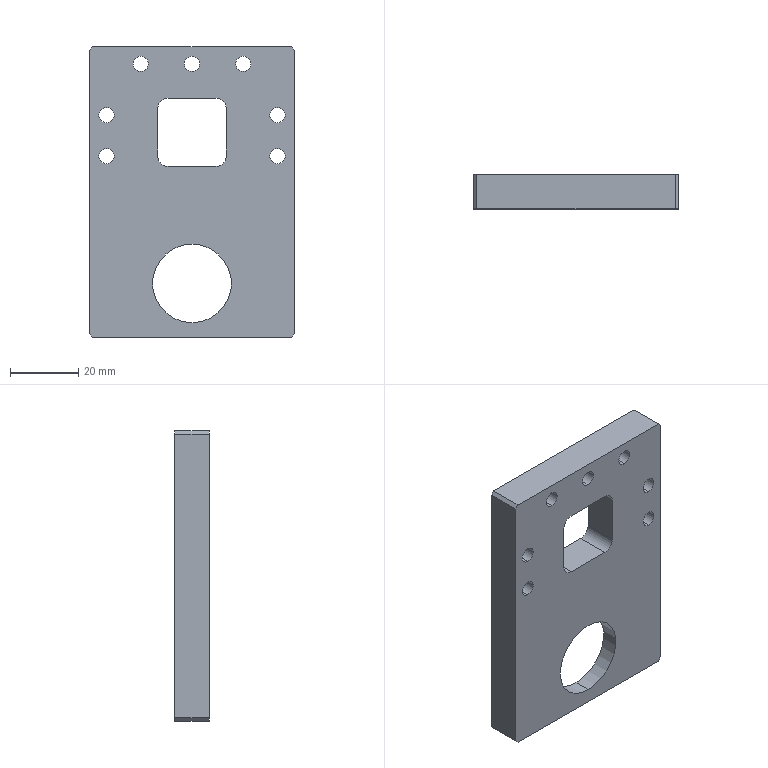Component | SolidWorks | CCDJSLiftingCylinderFixingPlate02-1 | 1 solid | 61 faces | box 60 x 10 x 85 mm | volume 33588 mm3 | cylinder 36 | plane 25 | commonest cylinder face diameters 8 x14 4.5 x14 6 x6 23 x2
build123d program:
from build123d import *

# Parameters (mm, degrees)
SKETCH1_W                                       = 85
SKETCH1_H                                       = 60
BOSS_EXTRUDE1_DEPTH                             = 10
SKETCH2_W                                       = 20
SKETCH2_H                                       = 20
CUT_EXTRUDE1_DEPTH                              = 24
FILLET1_R                                       = 3
SKETCH3_W                                       = 42
SKETCH3_H                                       = 5
CUT_EXTRUDE2_DEPTH                              = 65
SKETCH4_R                                       = 11.5
CUT_EXTRUDE3_DEPTH                              = 65
SKETCH5_W                                       = 42
SKETCH5_H                                       = 8
BOSS_EXTRUDE2_DEPTH                             = 5
FILLET2_R                                       = 3
M4_HEX_SOCKET_HEAD_CAP_SCREW_CBORE1_D           = 4.5
M4_HEX_SOCKET_HEAD_CAP_SCREW_CBORE1_DEPTH       = 10.1
M4_HEX_SOCKET_HEAD_CAP_SCREW_CBORE1_CBORE_D     = 8
M4_HEX_SOCKET_HEAD_CAP_SCREW_CBORE1_CBORE_DEPTH = 4.4
M4_HEX_SOCKET_HEAD_CAP_SCREW_CBORE1_TIP         = 1.352
CHAMFER1_SIZE                                   = 1


with BuildPart() as part:
    # Sketch1 → Boss-Extrude1 (new body)
    with BuildSketch(Plane.XY):
        Rectangle(SKETCH1_W, SKETCH1_H)
    extrude(amount=BOSS_EXTRUDE1_DEPTH)

    # Sketch2 → Cut-Extrude1 (cut)
    with BuildSketch(Plane(origin=(0, 0, 0), x_dir=(-1, 0, 0), z_dir=(0, 0, -1))):
        with Locations((17.5, 0)):
            Rectangle(SKETCH2_W, SKETCH2_H)
    extrude(amount=-CUT_EXTRUDE1_DEPTH, mode=Mode.SUBTRACT)

    # Fillet1
    fillet1_edges = [part.edges().sort_by_distance(p)[0] for p in [
        (-7.5, -10, 5),
        (-7.5, 10, 5),
        (-27.5, 10, 5),
        (-27.5, -10, 5),
    ]]
    fillet(fillet1_edges, radius=FILLET1_R)

    # Sketch3 → Cut-Extrude2 (cut)
    with BuildSketch(Plane(origin=(0, 30, 0), x_dir=(1, 0, 0), z_dir=(0, 1, 0))):
        with Locations((21.5, -2.5)):
            Rectangle(SKETCH3_W, SKETCH3_H)
    extrude(amount=-CUT_EXTRUDE2_DEPTH, mode=Mode.SUBTRACT)

    # Sketch4 → Cut-Extrude3 (cut)
    with BuildSketch(Plane(origin=(0, 0, 5), x_dir=(-1, 0, 0), z_dir=(0, 0, -1))):
        with Locations((-26.75, 0)):
            Circle(SKETCH4_R)
    extrude(amount=-CUT_EXTRUDE3_DEPTH, mode=Mode.SUBTRACT)

    # Sketch5 → Boss-Extrude2 (add)
    with BuildSketch(Plane(origin=(0, 0, 5), x_dir=(-1, 0, 0), z_dir=(0, 0, -1))):
        with Locations((-21.5, 26)):
            Rectangle(SKETCH5_W, SKETCH5_H)
        with Locations((-21.5, -26)):
            Rectangle(SKETCH5_W, SKETCH5_H)
    extrude(amount=BOSS_EXTRUDE2_DEPTH)

    # Fillet2
    fillet2_edges = [part.edges().sort_by_distance(p)[0] for p in [
        (0.5, 22, 2.5),
        (0.5, -22, 2.5),
    ]]
    fillet(fillet2_edges, radius=FILLET2_R)

    # M4 Hex Socket Head Cap Screw CBORE1
    with Locations(Plane(origin=(0, 0, 0), x_dir=(-1, 0, 0), z_dir=(0, 0, -1))):
        with Locations((22.5, 25), (10.5, 25), (10.5, -25), (22.5, -25), (37.5, 0), (37.5, -15), (37.5, 15)):
            CounterBoreHole(M4_HEX_SOCKET_HEAD_CAP_SCREW_CBORE1_D / 2, M4_HEX_SOCKET_HEAD_CAP_SCREW_CBORE1_CBORE_D / 2, M4_HEX_SOCKET_HEAD_CAP_SCREW_CBORE1_CBORE_DEPTH, depth=M4_HEX_SOCKET_HEAD_CAP_SCREW_CBORE1_DEPTH)
            with Locations((0, 0, -(M4_HEX_SOCKET_HEAD_CAP_SCREW_CBORE1_DEPTH + M4_HEX_SOCKET_HEAD_CAP_SCREW_CBORE1_TIP / 2))):  # 118° drill point
                Cone(0, M4_HEX_SOCKET_HEAD_CAP_SCREW_CBORE1_D / 2, M4_HEX_SOCKET_HEAD_CAP_SCREW_CBORE1_TIP, mode=Mode.SUBTRACT)

    # Chamfer1
    chamfer1_edges = [part.edges().sort_by_distance(p)[0] for p in [
        (42.5, -30, 5),
        (-42.5, -30, 5),
        (-42.5, 30, 5),
        (42.5, 30, 5),
    ]]
    chamfer(chamfer1_edges, length=CHAMFER1_SIZE)


solid = part.part

# Placed as in the assembly
solid = solid.moved(Location((-159, 536.564, -101.07), (90, 0, -90)))